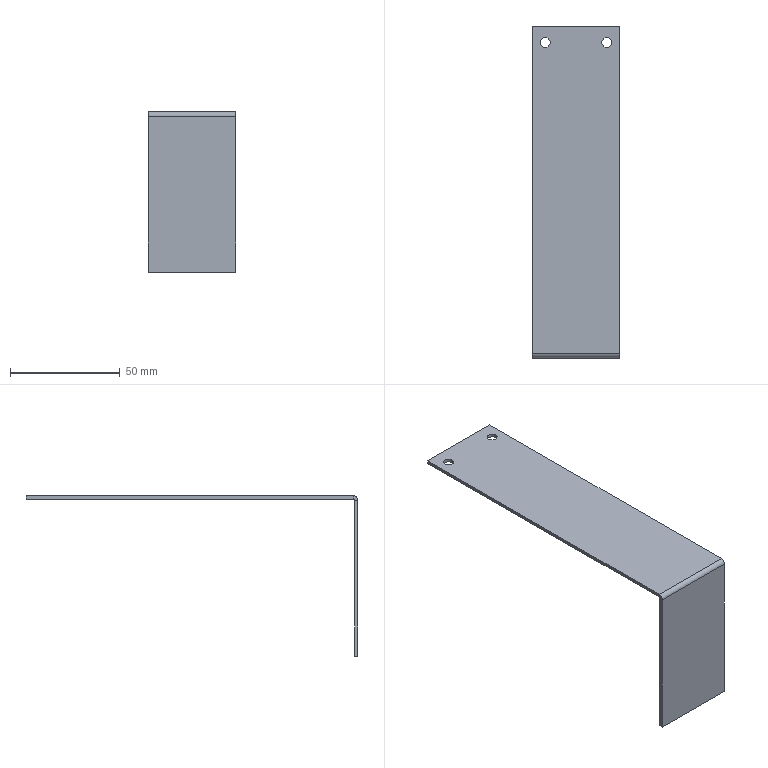Component | SolidWorks | A0117-1 | 1 solid | 18 faces | box 40 x 151 x 73 mm | volume 13270 mm3 | plane 12 | cylinder 6 | commonest cylinder face diameters 4.5 x4 4 x1 1 x1
STEP:
#1=CARTESIAN_POINT('',(0.5563,1.26,4.843));
#2=VERTEX_POINT('',#1);
#3=CARTESIAN_POINT('',(0.3792,1.26,4.843));
#4=VERTEX_POINT('',#3);
#5=CARTESIAN_POINT('',(0.4677,1.26,4.843));
#6=DIRECTION('',(0.,-0.,1.));
#7=DIRECTION('',(0.,-1.,0.));
#8=AXIS2_PLACEMENT_3D('',#5,#6,#7);
#9=CIRCLE('',#8,0.08858);
#10=EDGE_CURVE('',#2,#4,#9,.T.);
#11=ORIENTED_EDGE('',*,*,#10,.T.);
#12=CARTESIAN_POINT('',(0.3792,1.26,4.783));
#13=VERTEX_POINT('',#12);
#14=CARTESIAN_POINT('',(0.3792,1.26,4.783));
#15=DIRECTION('',(-0.,0.,-1.));
#16=VECTOR('',#15,39.37);
#17=LINE('',#14,#16);
#18=EDGE_CURVE('',#4,#13,#17,.T.);
#19=ORIENTED_EDGE('',*,*,#18,.T.);
#20=CARTESIAN_POINT('',(0.5563,1.26,4.783));
#21=VERTEX_POINT('',#20);
#22=CARTESIAN_POINT('',(0.4677,1.26,4.783));
#23=DIRECTION('',(-0.,0.,-1.));
#24=DIRECTION('',(1.,0.,0.));
#25=AXIS2_PLACEMENT_3D('',#22,#23,#24);
#26=CIRCLE('',#25,0.08858);
#27=EDGE_CURVE('',#13,#21,#26,.T.);
#28=ORIENTED_EDGE('',*,*,#27,.T.);
#29=CARTESIAN_POINT('',(0.5563,1.26,4.783));
#30=DIRECTION('',(-0.,0.,-1.));
#31=VECTOR('',#30,39.37);
#32=LINE('',#29,#31);
#33=EDGE_CURVE('',#2,#21,#32,.T.);
#34=ORIENTED_EDGE('',*,*,#33,.F.);
#35=EDGE_LOOP('',(#11,#19,#28,#34));
#36=FACE_OUTER_BOUND('',#35,.T.);
#37=CARTESIAN_POINT('',(0.4677,1.26,4.783));
#38=DIRECTION('',(-0.,0.,-1.));
#39=DIRECTION('',(1.,0.,0.));
#40=AXIS2_PLACEMENT_3D('',#37,#38,#39);
#41=CYLINDRICAL_SURFACE('',#40,0.08858);
#42=ADVANCED_FACE('',(#36),#41,.F.);
#43=CARTESIAN_POINT('',(1.659,1.26,4.843));
#44=VERTEX_POINT('',#43);
#45=CARTESIAN_POINT('',(1.482,1.26,4.843));
#46=VERTEX_POINT('',#45);
#47=CARTESIAN_POINT('',(1.57,1.26,4.843));
#48=DIRECTION('',(0.,-0.,1.));
#49=DIRECTION('',(0.,-1.,0.));
#50=AXIS2_PLACEMENT_3D('',#47,#48,#49);
#51=CIRCLE('',#50,0.08858);
#52=EDGE_CURVE('',#44,#46,#51,.T.);
#53=ORIENTED_EDGE('',*,*,#52,.T.);
#54=CARTESIAN_POINT('',(1.482,1.26,4.783));
#55=VERTEX_POINT('',#54);
#56=CARTESIAN_POINT('',(1.482,1.26,4.783));
#57=DIRECTION('',(-0.,0.,-1.));
#58=VECTOR('',#57,39.37);
#59=LINE('',#56,#58);
#60=EDGE_CURVE('',#46,#55,#59,.T.);
#61=ORIENTED_EDGE('',*,*,#60,.T.);
#62=CARTESIAN_POINT('',(1.659,1.26,4.783));
#63=VERTEX_POINT('',#62);
#64=CARTESIAN_POINT('',(1.57,1.26,4.783));
#65=DIRECTION('',(-0.,0.,-1.));
#66=DIRECTION('',(1.,0.,0.));
#67=AXIS2_PLACEMENT_3D('',#64,#65,#66);
#68=CIRCLE('',#67,0.08858);
#69=EDGE_CURVE('',#55,#63,#68,.T.);
#70=ORIENTED_EDGE('',*,*,#69,.T.);
#71=CARTESIAN_POINT('',(1.659,1.26,4.783));
#72=DIRECTION('',(-0.,0.,-1.));
#73=VECTOR('',#72,39.37);
#74=LINE('',#71,#73);
#75=EDGE_CURVE('',#44,#63,#74,.T.);
#76=ORIENTED_EDGE('',*,*,#75,.F.);
#77=EDGE_LOOP('',(#53,#61,#70,#76));
#78=FACE_OUTER_BOUND('',#77,.T.);
#79=CARTESIAN_POINT('',(1.57,1.26,4.783));
#80=DIRECTION('',(-0.,0.,-1.));
#81=DIRECTION('',(1.,0.,0.));
#82=AXIS2_PLACEMENT_3D('',#79,#80,#81);
#83=CYLINDRICAL_SURFACE('',#82,0.08858);
#84=ADVANCED_FACE('',(#78),#83,.F.);
#85=CARTESIAN_POINT('',(1.57,1.26,4.783));
#86=DIRECTION('',(-0.,0.,-1.));
#87=DIRECTION('',(1.,0.,0.));
#88=AXIS2_PLACEMENT_3D('',#85,#86,#87);
#89=CIRCLE('',#88,0.08858);
#90=EDGE_CURVE('',#63,#55,#89,.T.);
#91=ORIENTED_EDGE('',*,*,#90,.F.);
#92=ORIENTED_EDGE('',*,*,#69,.F.);
#93=EDGE_LOOP('',(#91,#92));
#94=FACE_BOUND('',#93,.T.);
#95=CARTESIAN_POINT('',(0.2315,-4.311,4.783));
#96=VERTEX_POINT('',#95);
#97=CARTESIAN_POINT('',(0.2315,1.555,4.783));
#98=VERTEX_POINT('',#97);
#99=CARTESIAN_POINT('',(0.2315,-4.39,4.783));
#100=DIRECTION('',(-0.,1.,0.));
#101=VECTOR('',#100,39.37);
#102=LINE('',#99,#101);
#103=EDGE_CURVE('',#96,#98,#102,.T.);
#104=ORIENTED_EDGE('',*,*,#103,.T.);
#105=CARTESIAN_POINT('',(1.806,1.555,4.783));
#106=VERTEX_POINT('',#105);
#107=CARTESIAN_POINT('',(1.806,1.555,4.783));
#108=DIRECTION('',(-1.,-0.,0.));
#109=VECTOR('',#108,39.37);
#110=LINE('',#107,#109);
#111=EDGE_CURVE('',#106,#98,#110,.T.);
#112=ORIENTED_EDGE('',*,*,#111,.F.);
#113=CARTESIAN_POINT('',(1.806,-4.311,4.783));
#114=VERTEX_POINT('',#113);
#115=CARTESIAN_POINT('',(1.806,-4.39,4.783));
#116=DIRECTION('',(-0.,1.,0.));
#117=VECTOR('',#116,39.37);
#118=LINE('',#115,#117);
#119=EDGE_CURVE('',#114,#106,#118,.T.);
#120=ORIENTED_EDGE('',*,*,#119,.F.);
#121=CARTESIAN_POINT('',(1.806,-4.311,4.783));
#122=DIRECTION('',(-1.,-0.,0.));
#123=VECTOR('',#122,39.37);
#124=LINE('',#121,#123);
#125=EDGE_CURVE('',#114,#96,#124,.T.);
#126=ORIENTED_EDGE('',*,*,#125,.T.);
#127=EDGE_LOOP('',(#104,#112,#120,#126));
#128=FACE_OUTER_BOUND('',#127,.T.);
#129=CARTESIAN_POINT('',(0.4677,1.26,4.783));
#130=DIRECTION('',(-0.,0.,-1.));
#131=DIRECTION('',(1.,0.,0.));
#132=AXIS2_PLACEMENT_3D('',#129,#130,#131);
#133=CIRCLE('',#132,0.08858);
#134=EDGE_CURVE('',#21,#13,#133,.T.);
#135=ORIENTED_EDGE('',*,*,#134,.F.);
#136=ORIENTED_EDGE('',*,*,#27,.F.);
#137=EDGE_LOOP('',(#135,#136));
#138=FACE_BOUND('',#137,.T.);
#139=CARTESIAN_POINT('',(1.806,-4.39,4.783));
#140=DIRECTION('',(0.,-0.,1.));
#141=DIRECTION('',(0.,-1.,-0.));
#142=AXIS2_PLACEMENT_3D('',#139,#140,#141);
#143=PLANE('',#142);
#144=ADVANCED_FACE('',(#94,#128,#138),#143,.F.);
#145=CARTESIAN_POINT('',(1.806,-4.311,4.843));
#146=VERTEX_POINT('',#145);
#147=CARTESIAN_POINT('',(1.806,-4.311,4.843));
#148=DIRECTION('',(-0.,0.,-1.));
#149=VECTOR('',#148,39.37);
#150=LINE('',#147,#149);
#151=EDGE_CURVE('',#146,#114,#150,.T.);
#152=ORIENTED_EDGE('',*,*,#151,.F.);
#153=CARTESIAN_POINT('',(1.806,-4.39,4.764));
#154=VERTEX_POINT('',#153);
#155=CARTESIAN_POINT('',(1.806,-4.311,4.764));
#156=DIRECTION('',(-1.,-0.,0.));
#157=DIRECTION('',(0.,0.,1.));
#158=AXIS2_PLACEMENT_3D('',#155,#156,#157);
#159=CIRCLE('',#158,0.07874);
#160=EDGE_CURVE('',#154,#146,#159,.T.);
#161=ORIENTED_EDGE('',*,*,#160,.F.);
#162=CARTESIAN_POINT('',(1.806,-4.331,4.764));
#163=VERTEX_POINT('',#162);
#164=CARTESIAN_POINT('',(1.806,-4.331,4.764));
#165=DIRECTION('',(0.,-1.,-0.));
#166=VECTOR('',#165,39.37);
#167=LINE('',#164,#166);
#168=EDGE_CURVE('',#163,#154,#167,.T.);
#169=ORIENTED_EDGE('',*,*,#168,.F.);
#170=CARTESIAN_POINT('',(1.806,-4.311,4.764));
#171=DIRECTION('',(-1.,-0.,0.));
#172=DIRECTION('',(0.,0.,1.));
#173=AXIS2_PLACEMENT_3D('',#170,#171,#172);
#174=CIRCLE('',#173,0.01969);
#175=EDGE_CURVE('',#163,#114,#174,.T.);
#176=ORIENTED_EDGE('',*,*,#175,.T.);
#177=EDGE_LOOP('',(#152,#161,#169,#176));
#178=FACE_OUTER_BOUND('',#177,.T.);
#179=CARTESIAN_POINT('',(1.806,-4.311,4.843));
#180=DIRECTION('',(1.,0.,-0.));
#181=DIRECTION('',(0.,-0.,1.));
#182=AXIS2_PLACEMENT_3D('',#179,#180,#181);
#183=PLANE('',#182);
#184=ADVANCED_FACE('',(#178),#183,.T.);
#185=CARTESIAN_POINT('',(1.806,1.555,4.843));
#186=VERTEX_POINT('',#185);
#187=CARTESIAN_POINT('',(1.806,-4.39,4.843));
#188=DIRECTION('',(-0.,1.,0.));
#189=VECTOR('',#188,39.37);
#190=LINE('',#187,#189);
#191=EDGE_CURVE('',#146,#186,#190,.T.);
#192=ORIENTED_EDGE('',*,*,#191,.F.);
#193=ORIENTED_EDGE('',*,*,#151,.T.);
#194=ORIENTED_EDGE('',*,*,#119,.T.);
#195=CARTESIAN_POINT('',(1.806,1.555,4.843));
#196=DIRECTION('',(-0.,0.,-1.));
#197=VECTOR('',#196,39.37);
#198=LINE('',#195,#197);
#199=EDGE_CURVE('',#186,#106,#198,.T.);
#200=ORIENTED_EDGE('',*,*,#199,.F.);
#201=EDGE_LOOP('',(#192,#193,#194,#200));
#202=FACE_OUTER_BOUND('',#201,.T.);
#203=CARTESIAN_POINT('',(1.806,-4.331,4.764));
#204=DIRECTION('',(1.,0.,-0.));
#205=DIRECTION('',(0.,-0.,1.));
#206=AXIS2_PLACEMENT_3D('',#203,#204,#205);
#207=PLANE('',#206);
#208=ADVANCED_FACE('',(#202),#207,.T.);
#209=CARTESIAN_POINT('',(0.2315,-4.39,4.764));
#210=VERTEX_POINT('',#209);
#211=CARTESIAN_POINT('',(0.2315,-4.331,4.764));
#212=VERTEX_POINT('',#211);
#213=CARTESIAN_POINT('',(0.2315,-4.39,4.764));
#214=DIRECTION('',(-0.,1.,0.));
#215=VECTOR('',#214,39.37);
#216=LINE('',#213,#215);
#217=EDGE_CURVE('',#210,#212,#216,.T.);
#218=ORIENTED_EDGE('',*,*,#217,.F.);
#219=CARTESIAN_POINT('',(0.2315,-4.311,4.843));
#220=VERTEX_POINT('',#219);
#221=CARTESIAN_POINT('',(0.2315,-4.311,4.764));
#222=DIRECTION('',(-1.,-0.,0.));
#223=DIRECTION('',(0.,0.,1.));
#224=AXIS2_PLACEMENT_3D('',#221,#222,#223);
#225=CIRCLE('',#224,0.07874);
#226=EDGE_CURVE('',#210,#220,#225,.T.);
#227=ORIENTED_EDGE('',*,*,#226,.T.);
#228=CARTESIAN_POINT('',(0.2315,-4.311,4.783));
#229=DIRECTION('',(0.,-0.,1.));
#230=VECTOR('',#229,39.37);
#231=LINE('',#228,#230);
#232=EDGE_CURVE('',#96,#220,#231,.T.);
#233=ORIENTED_EDGE('',*,*,#232,.F.);
#234=CARTESIAN_POINT('',(0.2315,-4.311,4.764));
#235=DIRECTION('',(-1.,-0.,0.));
#236=DIRECTION('',(0.,0.,1.));
#237=AXIS2_PLACEMENT_3D('',#234,#235,#236);
#238=CIRCLE('',#237,0.01969);
#239=EDGE_CURVE('',#212,#96,#238,.T.);
#240=ORIENTED_EDGE('',*,*,#239,.F.);
#241=EDGE_LOOP('',(#218,#227,#233,#240));
#242=FACE_OUTER_BOUND('',#241,.T.);
#243=CARTESIAN_POINT('',(0.2315,-4.39,4.764));
#244=DIRECTION('',(-1.,-0.,0.));
#245=DIRECTION('',(-0.,0.,-1.));
#246=AXIS2_PLACEMENT_3D('',#243,#244,#245);
#247=PLANE('',#246);
#248=ADVANCED_FACE('',(#242),#247,.T.);
#249=CARTESIAN_POINT('',(0.2315,-4.39,1.969));
#250=VERTEX_POINT('',#249);
#251=CARTESIAN_POINT('',(0.2315,-4.39,1.969));
#252=DIRECTION('',(0.,-0.,1.));
#253=VECTOR('',#252,39.37);
#254=LINE('',#251,#253);
#255=EDGE_CURVE('',#250,#210,#254,.T.);
#256=ORIENTED_EDGE('',*,*,#255,.T.);
#257=ORIENTED_EDGE('',*,*,#217,.T.);
#258=CARTESIAN_POINT('',(0.2315,-4.331,1.969));
#259=VERTEX_POINT('',#258);
#260=CARTESIAN_POINT('',(0.2315,-4.331,1.969));
#261=DIRECTION('',(0.,-0.,1.));
#262=VECTOR('',#261,39.37);
#263=LINE('',#260,#262);
#264=EDGE_CURVE('',#259,#212,#263,.T.);
#265=ORIENTED_EDGE('',*,*,#264,.F.);
#266=CARTESIAN_POINT('',(0.2315,-4.331,1.969));
#267=DIRECTION('',(0.,-1.,-0.));
#268=VECTOR('',#267,39.37);
#269=LINE('',#266,#268);
#270=EDGE_CURVE('',#259,#250,#269,.T.);
#271=ORIENTED_EDGE('',*,*,#270,.T.);
#272=EDGE_LOOP('',(#256,#257,#265,#271));
#273=FACE_OUTER_BOUND('',#272,.T.);
#274=CARTESIAN_POINT('',(0.2315,-4.311,4.783));
#275=DIRECTION('',(-1.,-0.,0.));
#276=DIRECTION('',(-0.,0.,-1.));
#277=AXIS2_PLACEMENT_3D('',#274,#275,#276);
#278=PLANE('',#277);
#279=ADVANCED_FACE('',(#273),#278,.T.);
#280=CARTESIAN_POINT('',(0.2315,1.555,4.843));
#281=VERTEX_POINT('',#280);
#282=CARTESIAN_POINT('',(0.2315,1.555,4.843));
#283=DIRECTION('',(-0.,0.,-1.));
#284=VECTOR('',#283,39.37);
#285=LINE('',#282,#284);
#286=EDGE_CURVE('',#281,#98,#285,.T.);
#287=ORIENTED_EDGE('',*,*,#286,.F.);
#288=CARTESIAN_POINT('',(1.806,1.555,4.843));
#289=DIRECTION('',(-1.,-0.,0.));
#290=VECTOR('',#289,39.37);
#291=LINE('',#288,#290);
#292=EDGE_CURVE('',#186,#281,#291,.T.);
#293=ORIENTED_EDGE('',*,*,#292,.F.);
#294=ORIENTED_EDGE('',*,*,#199,.T.);
#295=ORIENTED_EDGE('',*,*,#111,.T.);
#296=EDGE_LOOP('',(#287,#293,#294,#295));
#297=FACE_OUTER_BOUND('',#296,.T.);
#298=CARTESIAN_POINT('',(1.806,1.555,4.843));
#299=DIRECTION('',(-0.,1.,0.));
#300=DIRECTION('',(0.,-0.,1.));
#301=AXIS2_PLACEMENT_3D('',#298,#299,#300);
#302=PLANE('',#301);
#303=ADVANCED_FACE('',(#297),#302,.T.);
#304=ORIENTED_EDGE('',*,*,#10,.F.);
#305=CARTESIAN_POINT('',(0.4677,1.26,4.843));
#306=DIRECTION('',(0.,-0.,1.));
#307=DIRECTION('',(0.,-1.,0.));
#308=AXIS2_PLACEMENT_3D('',#305,#306,#307);
#309=CIRCLE('',#308,0.08858);
#310=EDGE_CURVE('',#4,#2,#309,.T.);
#311=ORIENTED_EDGE('',*,*,#310,.F.);
#312=EDGE_LOOP('',(#304,#311));
#313=FACE_BOUND('',#312,.T.);
#314=ORIENTED_EDGE('',*,*,#52,.F.);
#315=CARTESIAN_POINT('',(1.57,1.26,4.843));
#316=DIRECTION('',(0.,-0.,1.));
#317=DIRECTION('',(0.,-1.,0.));
#318=AXIS2_PLACEMENT_3D('',#315,#316,#317);
#319=CIRCLE('',#318,0.08858);
#320=EDGE_CURVE('',#46,#44,#319,.T.);
#321=ORIENTED_EDGE('',*,*,#320,.F.);
#322=EDGE_LOOP('',(#314,#321));
#323=FACE_BOUND('',#322,.T.);
#324=CARTESIAN_POINT('',(0.2315,-4.39,4.843));
#325=DIRECTION('',(-0.,1.,0.));
#326=VECTOR('',#325,39.37);
#327=LINE('',#324,#326);
#328=EDGE_CURVE('',#220,#281,#327,.T.);
#329=ORIENTED_EDGE('',*,*,#328,.F.);
#330=CARTESIAN_POINT('',(1.806,-4.311,4.843));
#331=DIRECTION('',(-1.,-0.,0.));
#332=VECTOR('',#331,39.37);
#333=LINE('',#330,#332);
#334=EDGE_CURVE('',#146,#220,#333,.T.);
#335=ORIENTED_EDGE('',*,*,#334,.F.);
#336=ORIENTED_EDGE('',*,*,#191,.T.);
#337=ORIENTED_EDGE('',*,*,#292,.T.);
#338=EDGE_LOOP('',(#329,#335,#336,#337));
#339=FACE_OUTER_BOUND('',#338,.T.);
#340=CARTESIAN_POINT('',(1.806,-4.39,4.843));
#341=DIRECTION('',(0.,-0.,1.));
#342=DIRECTION('',(0.,-1.,-0.));
#343=AXIS2_PLACEMENT_3D('',#340,#341,#342);
#344=PLANE('',#343);
#345=ADVANCED_FACE('',(#313,#323,#339),#344,.T.);
#346=ORIENTED_EDGE('',*,*,#226,.F.);
#347=CARTESIAN_POINT('',(1.806,-4.39,4.764));
#348=DIRECTION('',(-1.,-0.,0.));
#349=VECTOR('',#348,39.37);
#350=LINE('',#347,#349);
#351=EDGE_CURVE('',#154,#210,#350,.T.);
#352=ORIENTED_EDGE('',*,*,#351,.F.);
#353=ORIENTED_EDGE('',*,*,#160,.T.);
#354=ORIENTED_EDGE('',*,*,#334,.T.);
#355=EDGE_LOOP('',(#346,#352,#353,#354));
#356=FACE_OUTER_BOUND('',#355,.T.);
#357=CARTESIAN_POINT('',(1.806,-4.311,4.764));
#358=DIRECTION('',(-1.,-0.,0.));
#359=DIRECTION('',(0.,0.,-1.));
#360=AXIS2_PLACEMENT_3D('',#357,#358,#359);
#361=CYLINDRICAL_SURFACE('',#360,0.07874);
#362=ADVANCED_FACE('',(#356),#361,.T.);
#363=ORIENTED_EDGE('',*,*,#255,.F.);
#364=CARTESIAN_POINT('',(1.806,-4.39,1.969));
#365=VERTEX_POINT('',#364);
#366=CARTESIAN_POINT('',(1.806,-4.39,1.969));
#367=DIRECTION('',(-1.,-0.,0.));
#368=VECTOR('',#367,39.37);
#369=LINE('',#366,#368);
#370=EDGE_CURVE('',#365,#250,#369,.T.);
#371=ORIENTED_EDGE('',*,*,#370,.F.);
#372=CARTESIAN_POINT('',(1.806,-4.39,1.969));
#373=DIRECTION('',(0.,-0.,1.));
#374=VECTOR('',#373,39.37);
#375=LINE('',#372,#374);
#376=EDGE_CURVE('',#365,#154,#375,.T.);
#377=ORIENTED_EDGE('',*,*,#376,.T.);
#378=ORIENTED_EDGE('',*,*,#351,.T.);
#379=EDGE_LOOP('',(#363,#371,#377,#378));
#380=FACE_OUTER_BOUND('',#379,.T.);
#381=CARTESIAN_POINT('',(1.806,-4.39,1.969));
#382=DIRECTION('',(0.,-1.,-0.));
#383=DIRECTION('',(-0.,0.,-1.));
#384=AXIS2_PLACEMENT_3D('',#381,#382,#383);
#385=PLANE('',#384);
#386=ADVANCED_FACE('',(#380),#385,.T.);
#387=ORIENTED_EDGE('',*,*,#270,.F.);
#388=CARTESIAN_POINT('',(1.806,-4.331,1.969));
#389=VERTEX_POINT('',#388);
#390=CARTESIAN_POINT('',(1.806,-4.331,1.969));
#391=DIRECTION('',(-1.,-0.,0.));
#392=VECTOR('',#391,39.37);
#393=LINE('',#390,#392);
#394=EDGE_CURVE('',#389,#259,#393,.T.);
#395=ORIENTED_EDGE('',*,*,#394,.F.);
#396=CARTESIAN_POINT('',(1.806,-4.331,1.969));
#397=DIRECTION('',(0.,-1.,-0.));
#398=VECTOR('',#397,39.37);
#399=LINE('',#396,#398);
#400=EDGE_CURVE('',#389,#365,#399,.T.);
#401=ORIENTED_EDGE('',*,*,#400,.T.);
#402=ORIENTED_EDGE('',*,*,#370,.T.);
#403=EDGE_LOOP('',(#387,#395,#401,#402));
#404=FACE_OUTER_BOUND('',#403,.T.);
#405=CARTESIAN_POINT('',(1.806,-4.331,1.969));
#406=DIRECTION('',(-0.,0.,-1.));
#407=DIRECTION('',(1.,0.,-0.));
#408=AXIS2_PLACEMENT_3D('',#405,#406,#407);
#409=PLANE('',#408);
#410=ADVANCED_FACE('',(#404),#409,.T.);
#411=ORIENTED_EDGE('',*,*,#264,.T.);
#412=CARTESIAN_POINT('',(1.806,-4.331,4.764));
#413=DIRECTION('',(-1.,-0.,0.));
#414=VECTOR('',#413,39.37);
#415=LINE('',#412,#414);
#416=EDGE_CURVE('',#163,#212,#415,.T.);
#417=ORIENTED_EDGE('',*,*,#416,.F.);
#418=CARTESIAN_POINT('',(1.806,-4.331,1.969));
#419=DIRECTION('',(0.,-0.,1.));
#420=VECTOR('',#419,39.37);
#421=LINE('',#418,#420);
#422=EDGE_CURVE('',#389,#163,#421,.T.);
#423=ORIENTED_EDGE('',*,*,#422,.F.);
#424=ORIENTED_EDGE('',*,*,#394,.T.);
#425=EDGE_LOOP('',(#411,#417,#423,#424));
#426=FACE_OUTER_BOUND('',#425,.T.);
#427=CARTESIAN_POINT('',(1.806,-4.331,1.969));
#428=DIRECTION('',(0.,-1.,-0.));
#429=DIRECTION('',(-0.,0.,-1.));
#430=AXIS2_PLACEMENT_3D('',#427,#428,#429);
#431=PLANE('',#430);
#432=ADVANCED_FACE('',(#426),#431,.F.);
#433=ORIENTED_EDGE('',*,*,#239,.T.);
#434=ORIENTED_EDGE('',*,*,#125,.F.);
#435=ORIENTED_EDGE('',*,*,#175,.F.);
#436=ORIENTED_EDGE('',*,*,#416,.T.);
#437=EDGE_LOOP('',(#433,#434,#435,#436));
#438=FACE_OUTER_BOUND('',#437,.T.);
#439=CARTESIAN_POINT('',(1.806,-4.311,4.764));
#440=DIRECTION('',(-1.,-0.,0.));
#441=DIRECTION('',(0.,0.,-1.));
#442=AXIS2_PLACEMENT_3D('',#439,#440,#441);
#443=CYLINDRICAL_SURFACE('',#442,0.01969);
#444=ADVANCED_FACE('',(#438),#443,.F.);
#445=ORIENTED_EDGE('',*,*,#422,.T.);
#446=ORIENTED_EDGE('',*,*,#168,.T.);
#447=ORIENTED_EDGE('',*,*,#376,.F.);
#448=ORIENTED_EDGE('',*,*,#400,.F.);
#449=EDGE_LOOP('',(#445,#446,#447,#448));
#450=FACE_OUTER_BOUND('',#449,.T.);
#451=CARTESIAN_POINT('',(1.806,-4.311,4.764));
#452=DIRECTION('',(1.,0.,-0.));
#453=DIRECTION('',(0.,-0.,1.));
#454=AXIS2_PLACEMENT_3D('',#451,#452,#453);
#455=PLANE('',#454);
#456=ADVANCED_FACE('',(#450),#455,.T.);
#457=ORIENTED_EDGE('',*,*,#103,.F.);
#458=ORIENTED_EDGE('',*,*,#232,.T.);
#459=ORIENTED_EDGE('',*,*,#328,.T.);
#460=ORIENTED_EDGE('',*,*,#286,.T.);
#461=EDGE_LOOP('',(#457,#458,#459,#460));
#462=FACE_OUTER_BOUND('',#461,.T.);
#463=CARTESIAN_POINT('',(0.2315,-4.311,4.764));
#464=DIRECTION('',(1.,0.,-0.));
#465=DIRECTION('',(0.,-0.,1.));
#466=AXIS2_PLACEMENT_3D('',#463,#464,#465);
#467=PLANE('',#466);
#468=ADVANCED_FACE('',(#462),#467,.F.);
#469=ORIENTED_EDGE('',*,*,#60,.F.);
#470=ORIENTED_EDGE('',*,*,#320,.T.);
#471=ORIENTED_EDGE('',*,*,#75,.T.);
#472=ORIENTED_EDGE('',*,*,#90,.T.);
#473=EDGE_LOOP('',(#469,#470,#471,#472));
#474=FACE_OUTER_BOUND('',#473,.T.);
#475=CARTESIAN_POINT('',(1.57,1.26,4.783));
#476=DIRECTION('',(-0.,0.,-1.));
#477=DIRECTION('',(1.,0.,0.));
#478=AXIS2_PLACEMENT_3D('',#475,#476,#477);
#479=CYLINDRICAL_SURFACE('',#478,0.08858);
#480=ADVANCED_FACE('',(#474),#479,.F.);
#481=ORIENTED_EDGE('',*,*,#18,.F.);
#482=ORIENTED_EDGE('',*,*,#310,.T.);
#483=ORIENTED_EDGE('',*,*,#33,.T.);
#484=ORIENTED_EDGE('',*,*,#134,.T.);
#485=EDGE_LOOP('',(#481,#482,#483,#484));
#486=FACE_OUTER_BOUND('',#485,.T.);
#487=CARTESIAN_POINT('',(0.4677,1.26,4.783));
#488=DIRECTION('',(-0.,0.,-1.));
#489=DIRECTION('',(1.,0.,0.));
#490=AXIS2_PLACEMENT_3D('',#487,#488,#489);
#491=CYLINDRICAL_SURFACE('',#490,0.08858);
#492=ADVANCED_FACE('',(#486),#491,.F.);
#493=CLOSED_SHELL('',(#42,#84,#144,#184,#208,#248,#279,#303,#345,#362,#386,#410,#432,#444,#456,#468,#480,#492));
#494=MANIFOLD_SOLID_BREP('',#493);
#495=CARTESIAN_POINT('',(0.,0.,0.));
#496=DIRECTION('',(0.,0.,1.));
#497=DIRECTION('',(1.,0.,0.));
#498=AXIS2_PLACEMENT_3D('',#495,#496,#497);
#499=(LENGTH_UNIT()NAMED_UNIT(*)SI_UNIT($,.METRE.));
#500=LENGTH_MEASURE_WITH_UNIT(LENGTH_MEASURE(0.0254),#499);
#501=DIMENSIONAL_EXPONENTS(1.,0.,0.,0.,0.,0.,0.);
#502=(CONVERSION_BASED_UNIT('',#500)LENGTH_UNIT()NAMED_UNIT(#501));
#503=UNCERTAINTY_MEASURE_WITH_UNIT(LENGTH_MEASURE(0.00001),#502,'','');
#504=(NAMED_UNIT(*)PLANE_ANGLE_UNIT()SI_UNIT($,.RADIAN.));
#505=(NAMED_UNIT(*)SI_UNIT($,.STERADIAN.)SOLID_ANGLE_UNIT());
#506=(GEOMETRIC_REPRESENTATION_CONTEXT(3)GLOBAL_UNCERTAINTY_ASSIGNED_CONTEXT((#503))GLOBAL_UNIT_ASSIGNED_CONTEXT((#502,#504,#505))REPRESENTATION_CONTEXT('',''));
#507=ADVANCED_BREP_SHAPE_REPRESENTATION('',(#494,#498),#506);
#508=COLOUR_RGB('',0.7922,0.8196,0.9333);
#509=FILL_AREA_STYLE_COLOUR('',#508);
#510=FILL_AREA_STYLE('',(#509));
#511=SURFACE_STYLE_FILL_AREA(#510);
#512=SURFACE_SIDE_STYLE('',(#511));
#513=SURFACE_STYLE_USAGE(.BOTH.,#512);
#514=PRESENTATION_STYLE_ASSIGNMENT((#513));
#515=STYLED_ITEM('',(#514),#494);
#516=PRESENTATION_LAYER_ASSIGNMENT('','',(#515));
#517=(LENGTH_UNIT()NAMED_UNIT(*)SI_UNIT($,.METRE.));
#518=LENGTH_MEASURE_WITH_UNIT(LENGTH_MEASURE(0.0254),#517);
#519=DIMENSIONAL_EXPONENTS(1.,0.,0.,0.,0.,0.,0.);
#520=(CONVERSION_BASED_UNIT('',#518)LENGTH_UNIT()NAMED_UNIT(#519));
#521=UNCERTAINTY_MEASURE_WITH_UNIT(LENGTH_MEASURE(0.00001),#520,'','');
#522=(NAMED_UNIT(*)PLANE_ANGLE_UNIT()SI_UNIT($,.RADIAN.));
#523=(NAMED_UNIT(*)SI_UNIT($,.STERADIAN.)SOLID_ANGLE_UNIT());
#524=(GEOMETRIC_REPRESENTATION_CONTEXT(3)GLOBAL_UNCERTAINTY_ASSIGNED_CONTEXT((#521))GLOBAL_UNIT_ASSIGNED_CONTEXT((#520,#522,#523))REPRESENTATION_CONTEXT('',''));
#525=MECHANICAL_DESIGN_GEOMETRIC_PRESENTATION_REPRESENTATION('',(#515),#524);